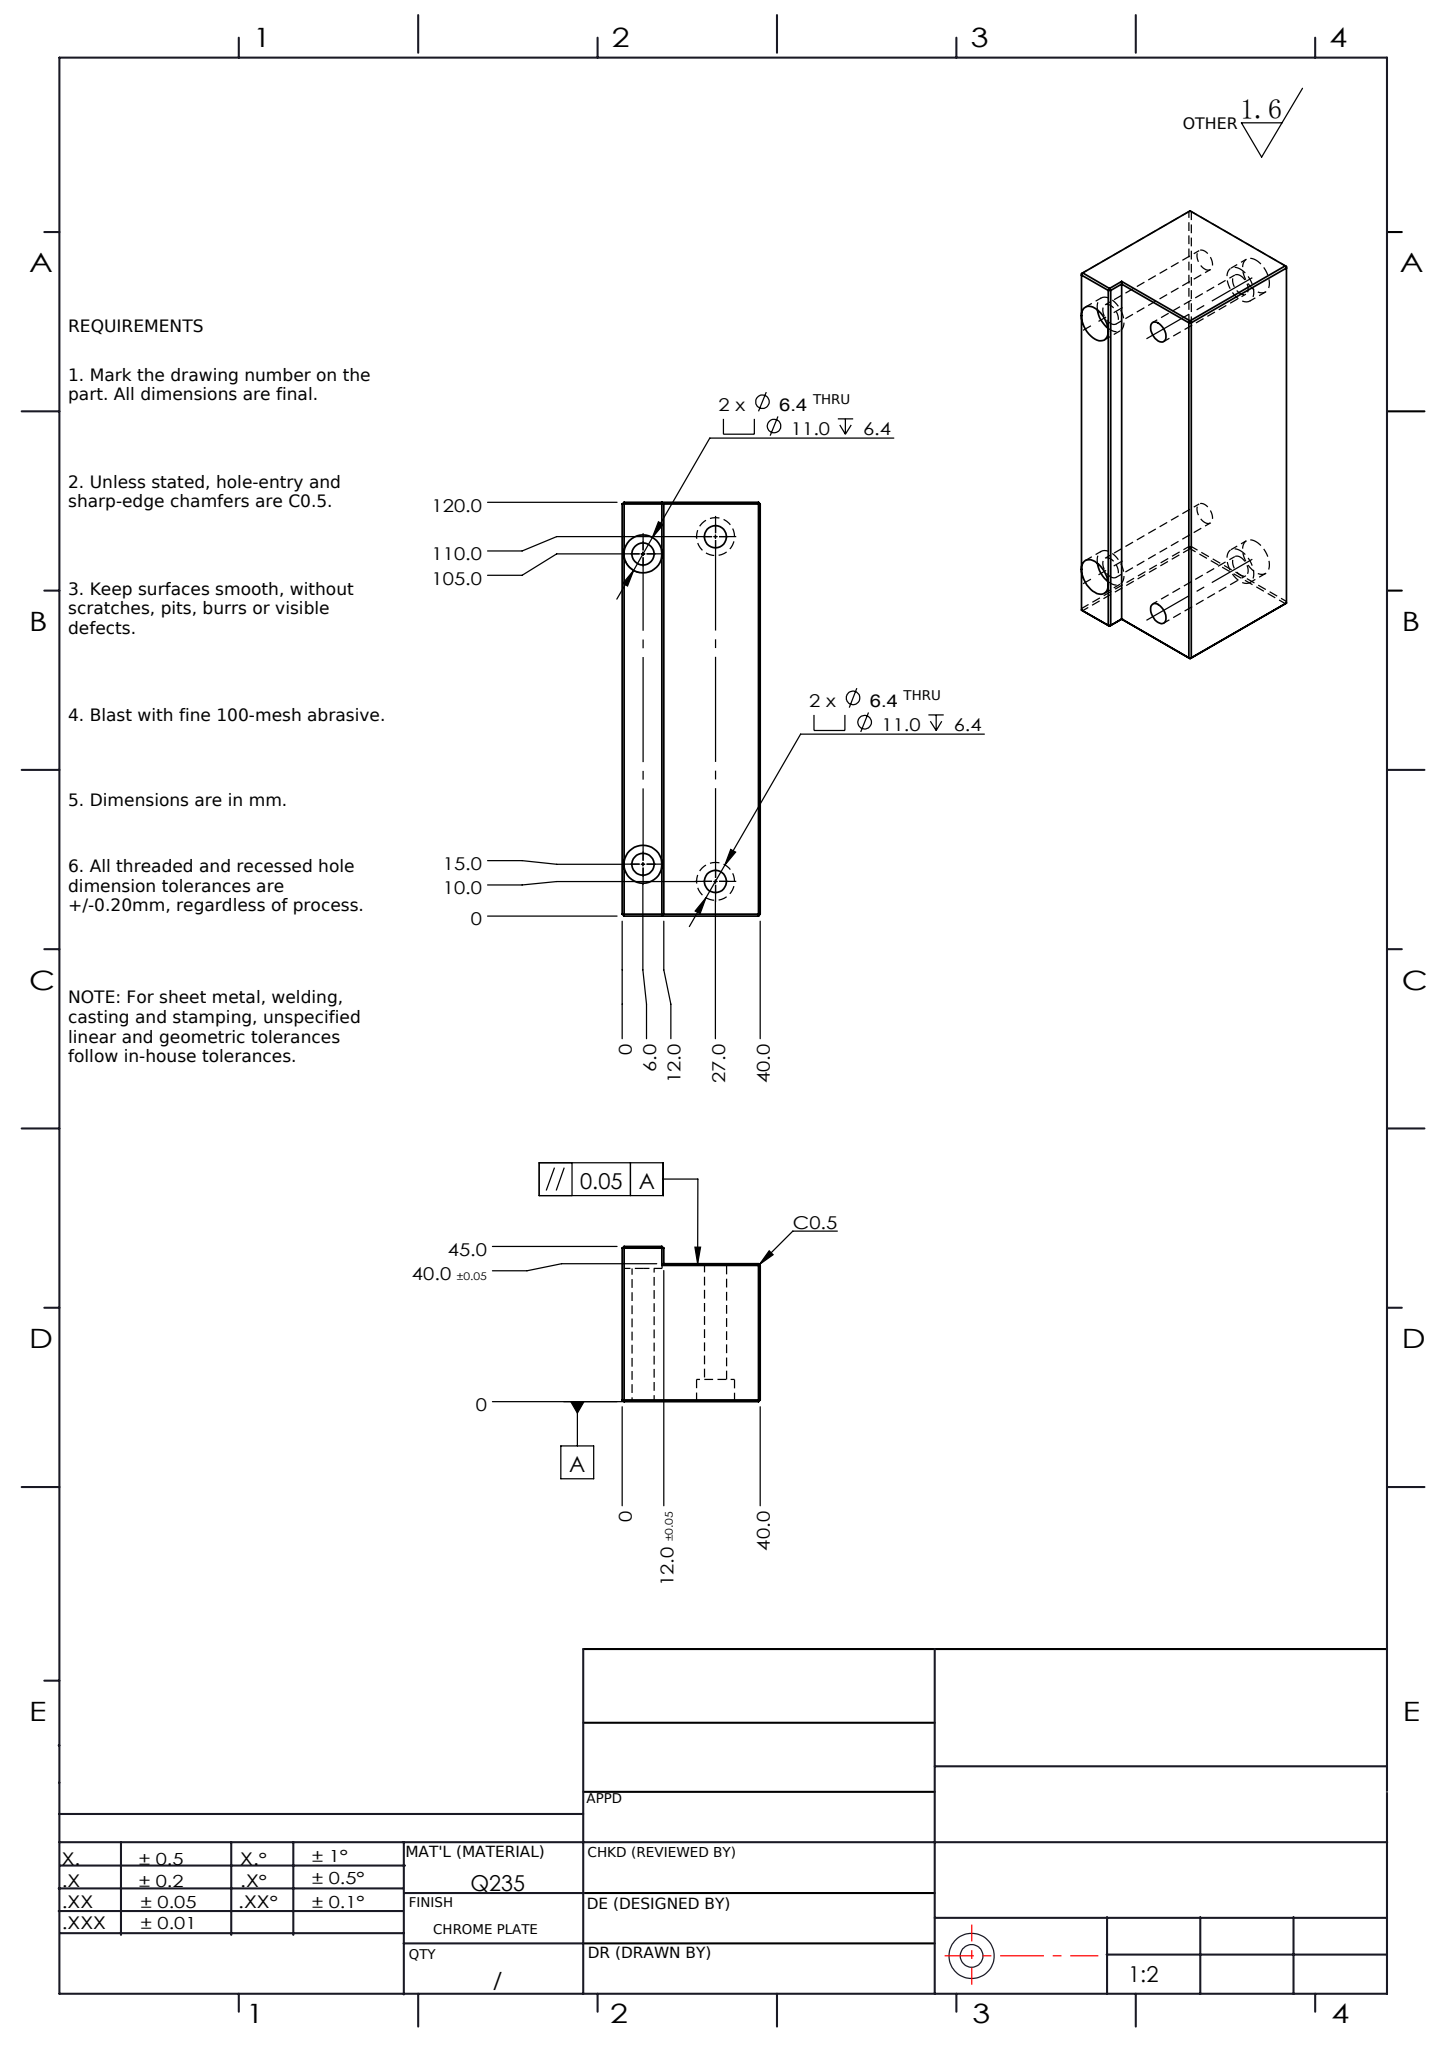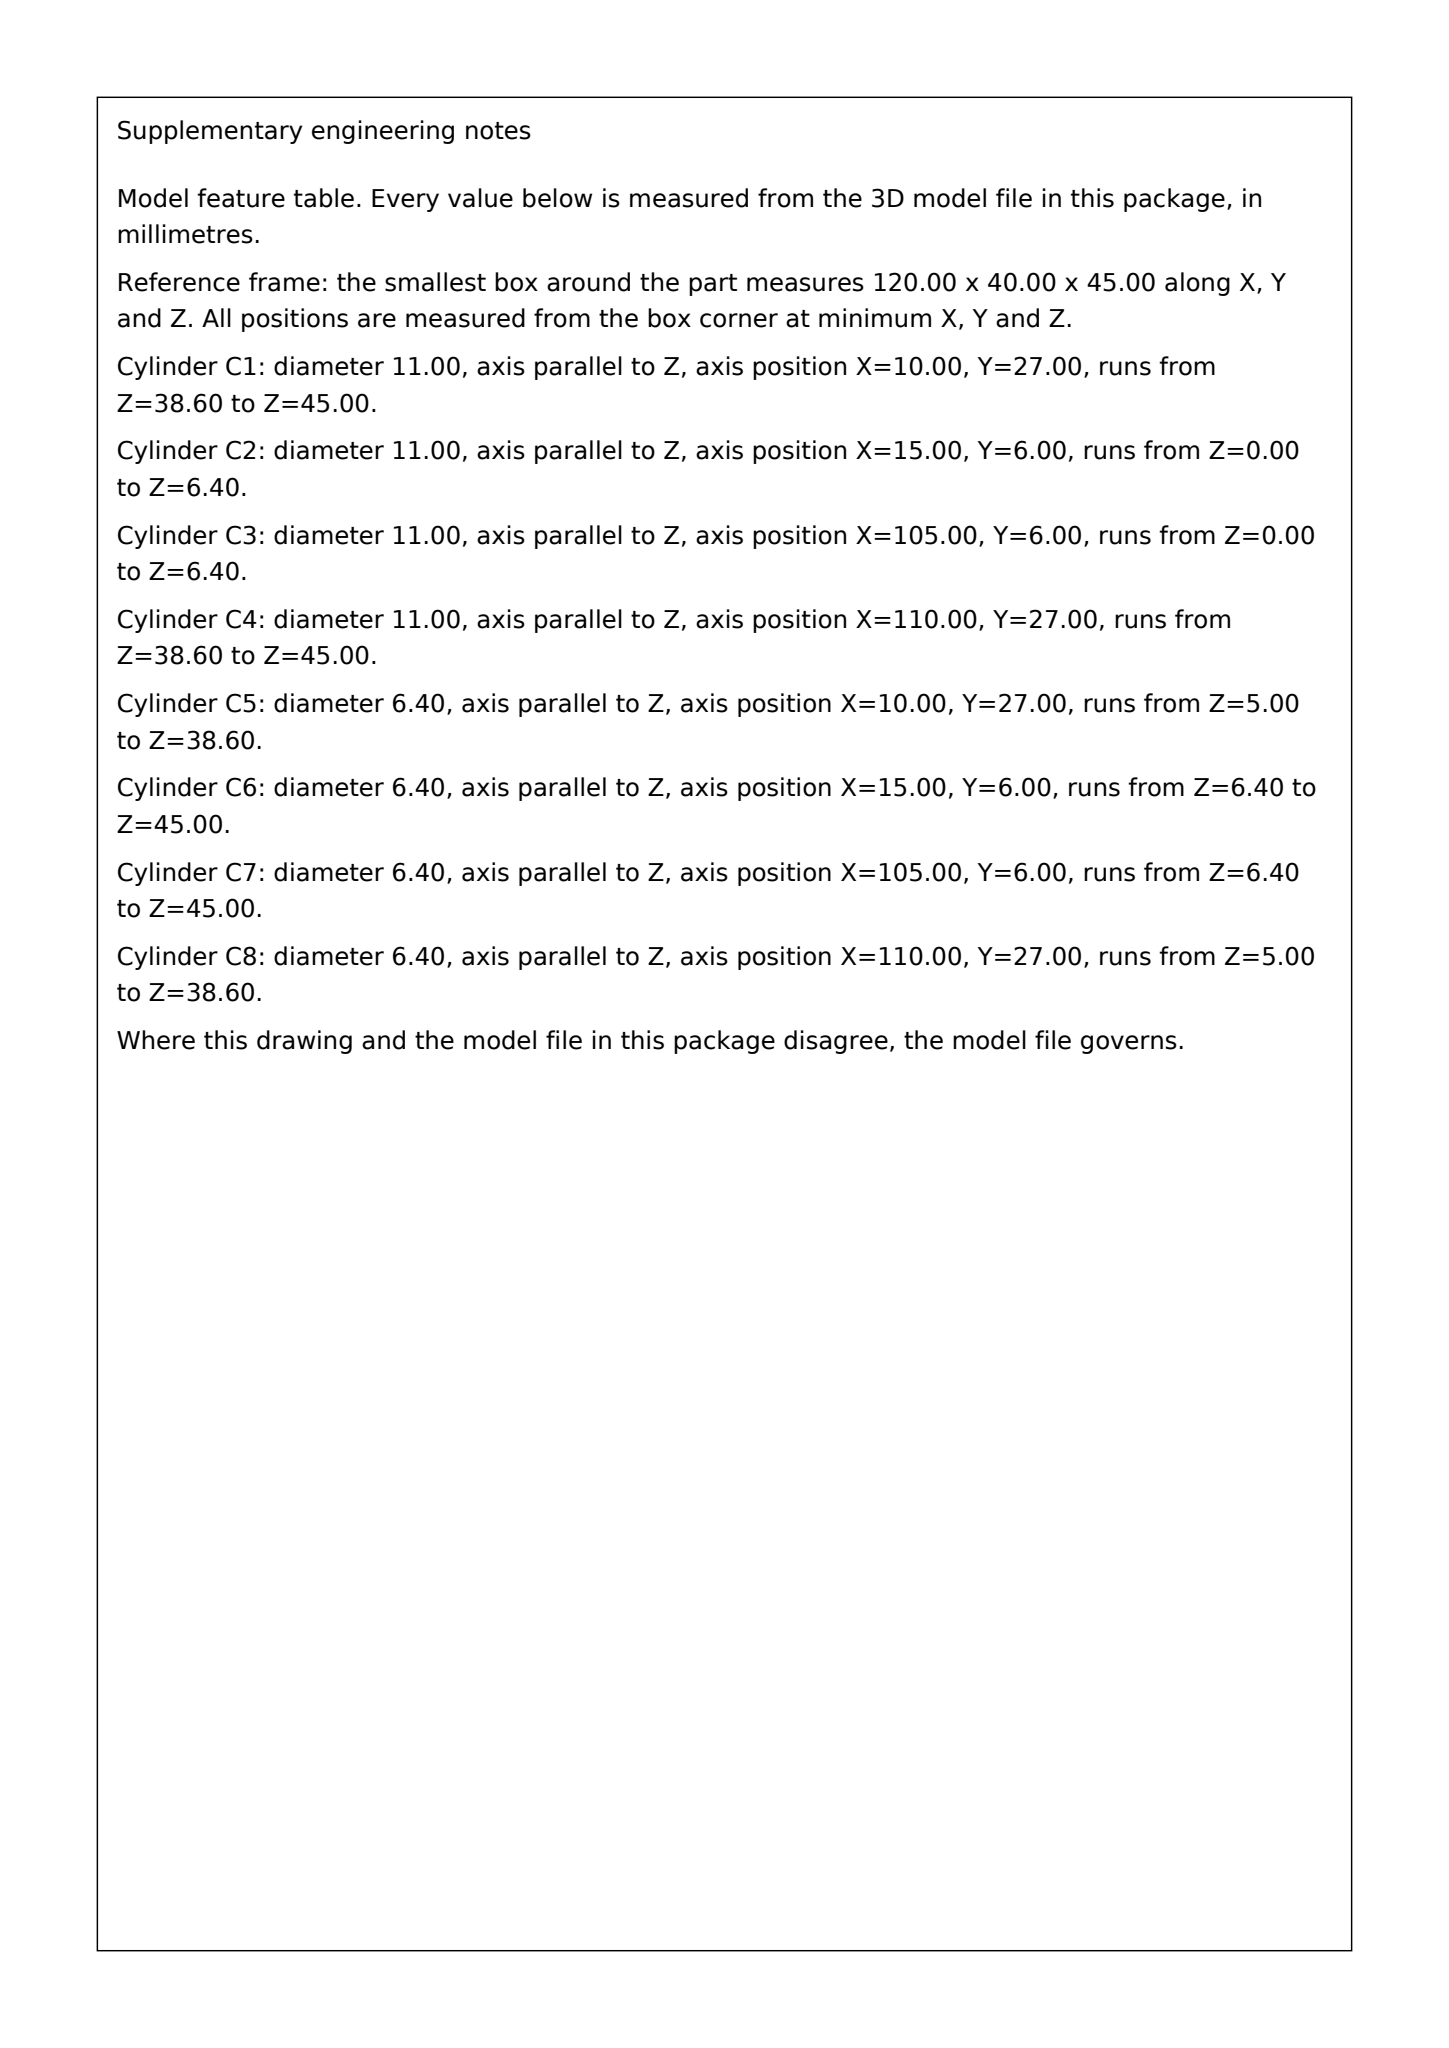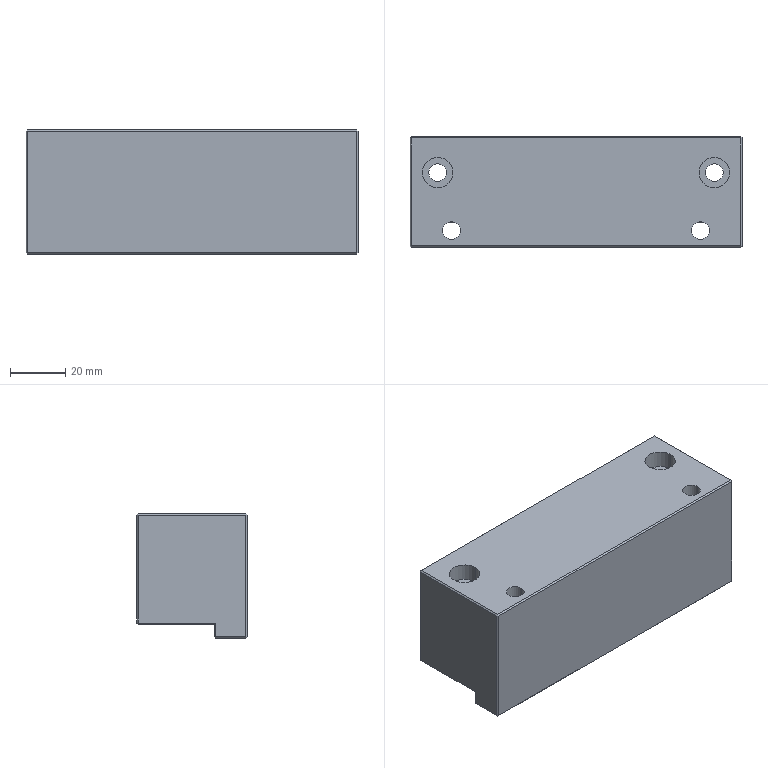Part | SolidWorks | mm | 1 solid | 57 faces | box 120 x 40 x 45 mm | volume 192005 mm3 | plane 41 | cylinder 16 | commonest cylinder face diameters 11 x8 6.4 x8